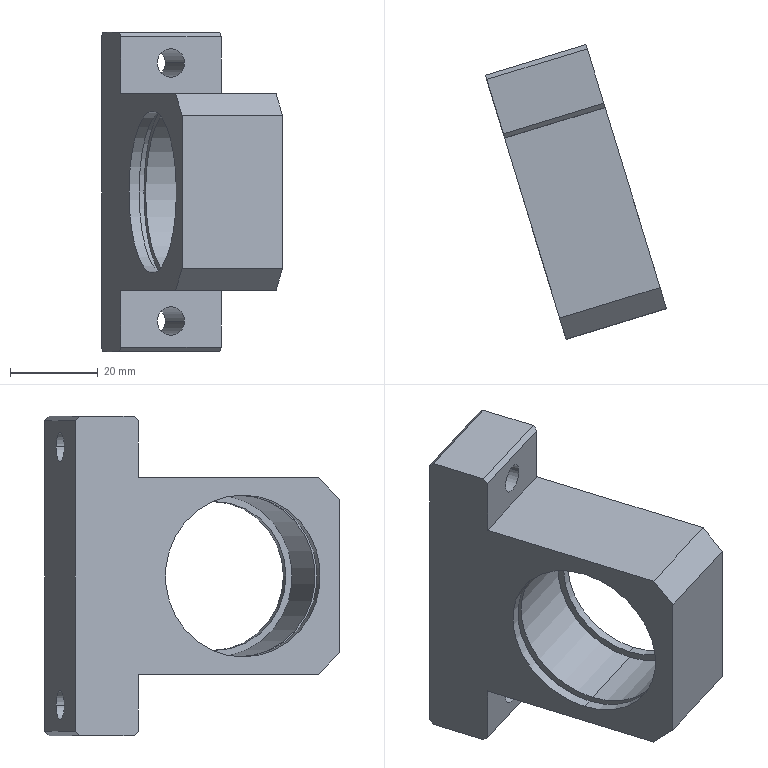Component | SolidWorks | v1ZHXTBGMWB6904ZZ_40SB1-1_V1ZHXTBearingMountingBaseSB1-1 | 1 solid | 31 faces | box 41.34 x 67.26 x 73 mm | volume 50736 mm3 | plane 19 | cylinder 12 | commonest cylinder face diameters 6.5 x4 37 x4 34 x2 39.8 x2
build123d program:
from build123d import *

# Parameters (mm, degrees)
BOSS_EXTRUDE1_DEPTH      = 12
BOSS_EXTRUDE1_DEPTH_BACK = 12
SKETCH3_R                = 3.25
CUT_EXTRUDE1_DEPTH       = 15
SKETCH4_R                = 3.25
CUT_EXTRUDE2_DEPTH       = 15
CHAMFER1_SIZE            = 5
CHAMFER2_SIZE            = 1


with BuildPart() as part:
    # Sketch1 → Boss-Extrude1 (new, two sides: drawn at the far end of the back side and taken through both)
    with BuildSketch(Plane.XY.offset(-BOSS_EXTRUDE1_DEPTH_BACK)):
        Polygon((-36.5, -40), (36.5, -40), (36.5, -25), (22.5, -25), (22.5, 23), (-22.5, 23), (-22.5, -25), (-36.5, -25), align=None)
    extrude(amount=BOSS_EXTRUDE1_DEPTH + BOSS_EXTRUDE1_DEPTH_BACK)

    # Sketch2 → Cut-Revolve1 (revolve, cut)
    with BuildSketch(Plane(origin=(0, 0, 0), x_dir=(0, 0, -1), z_dir=(1, 0, 0)), mode=Mode.PRIVATE) as cut_revolve1_sk:
        Polygon((-12, 0), (-12, 18.5), (-9.6, 18.5), (-9.6, 19.9), (-8, 19.9), (-8, 18.5), (10, 18.5), (10, 17), (12, 17), (12, 0), align=None)
    revolve(cut_revolve1_sk.sketch.rotate(Axis((0, 0, -12), (0, 0, 1)), 270), axis=Axis((0, 0, -12), (0, 0, 1)), mode=Mode.SUBTRACT)

    # Sketch3 → Cut-Extrude1 (cut)
    with BuildSketch(Plane(origin=(0, -40, 0), x_dir=(1, 0, 0), z_dir=(0, 1, 0))):
        with Locations(Location((-29.5, 0, 0), (0, 0, 270))):
            Circle(SKETCH3_R)
    extrude(amount=CUT_EXTRUDE1_DEPTH, mode=Mode.SUBTRACT)

    # Sketch4 → Cut-Extrude2 (cut)
    with BuildSketch(Plane(origin=(0, -40, 0), x_dir=(1, 0, 0), z_dir=(0, 1, 0))):
        with Locations(Location((29.5, 0, 0), (0, 0, 270))):
            Circle(SKETCH4_R)
    extrude(amount=CUT_EXTRUDE2_DEPTH, mode=Mode.SUBTRACT)

    # Chamfer1
    chamfer1_edges = [part.edges().sort_by_distance(p)[0] for p in [
        (-22.5, 23, 0),
        (22.5, 23, 0),
    ]]
    chamfer(chamfer1_edges, length=CHAMFER1_SIZE)

    # Chamfer2
    chamfer2_edges = [part.edges().sort_by_distance(p)[0] for p in [
        (-36.5, -25, 0),
        (36.5, -25, 0),
        (36.5, -40, 0),
        (-36.5, -40, 0),
    ]]
    chamfer(chamfer2_edges, length=CHAMFER2_SIZE)


solid = part.part

# Placed as in the assembly
solid = solid.moved(Location((165.24, -235.803, 375.239), (90, -73.032, -90)))
STEP:
#1=COLOUR_RGB('',0.7922,0.8196,0.9333);
#2=FILL_AREA_STYLE_COLOUR('',#1);
#3=FILL_AREA_STYLE('',(#2));
#4=SURFACE_STYLE_FILL_AREA(#3);
#5=SURFACE_SIDE_STYLE('',(#4));
#6=SURFACE_STYLE_USAGE(.BOTH.,#5);
#7=PRESENTATION_STYLE_ASSIGNMENT((#6));
#8=CARTESIAN_POINT('',(6.341,-8.305,13.612));
#9=VERTEX_POINT('',#8);
#10=CARTESIAN_POINT('',(6.096,-8.38,13.612));
#11=VERTEX_POINT('',#10);
#12=CARTESIAN_POINT('',(6.218,-8.342,13.612));
#13=DIRECTION('',(0.2918,-0.9565,-0.));
#14=DIRECTION('',(-0.9565,-0.2918,-0.));
#15=AXIS2_PLACEMENT_3D('',#12,#13,#14);
#16=CIRCLE('',#15,0.128);
#17=EDGE_CURVE('',#9,#11,#16,.T.);
#18=ORIENTED_EDGE('',*,*,#17,.T.);
#19=CARTESIAN_POINT('',(5.924,-7.815,13.612));
#20=VERTEX_POINT('',#19);
#21=CARTESIAN_POINT('',(6.096,-8.38,13.612));
#22=DIRECTION('',(-0.2918,0.9565,0.));
#23=VECTOR('',#22,39.37);
#24=LINE('',#21,#23);
#25=EDGE_CURVE('',#11,#20,#24,.T.);
#26=ORIENTED_EDGE('',*,*,#25,.T.);
#27=CARTESIAN_POINT('',(6.168,-7.74,13.612));
#28=VERTEX_POINT('',#27);
#29=CARTESIAN_POINT('',(6.046,-7.777,13.612));
#30=DIRECTION('',(0.2918,-0.9565,-0.));
#31=DIRECTION('',(-0.9565,-0.2918,-0.));
#32=AXIS2_PLACEMENT_3D('',#29,#30,#31);
#33=CIRCLE('',#32,0.128);
#34=EDGE_CURVE('',#28,#20,#33,.T.);
#35=ORIENTED_EDGE('',*,*,#34,.F.);
#36=CARTESIAN_POINT('',(6.341,-8.305,13.612));
#37=DIRECTION('',(-0.2918,0.9565,0.));
#38=VECTOR('',#37,39.37);
#39=LINE('',#36,#38);
#40=EDGE_CURVE('',#9,#28,#39,.T.);
#41=ORIENTED_EDGE('',*,*,#40,.F.);
#42=EDGE_LOOP('',(#18,#26,#35,#41));
#43=FACE_OUTER_BOUND('',#42,.T.);
#44=CARTESIAN_POINT('',(6.218,-8.342,13.612));
#45=DIRECTION('',(-0.2918,0.9565,0.));
#46=DIRECTION('',(0.9565,0.2918,0.));
#47=AXIS2_PLACEMENT_3D('',#44,#45,#46);
#48=CYLINDRICAL_SURFACE('',#47,0.128);
#49=ADVANCED_FACE('',(#43),#48,.F.);
#50=CARTESIAN_POINT('',(6.341,-8.305,15.935));
#51=VERTEX_POINT('',#50);
#52=CARTESIAN_POINT('',(6.096,-8.38,15.935));
#53=VERTEX_POINT('',#52);
#54=CARTESIAN_POINT('',(6.218,-8.342,15.935));
#55=DIRECTION('',(0.2918,-0.9565,-0.));
#56=DIRECTION('',(-0.9565,-0.2918,-0.));
#57=AXIS2_PLACEMENT_3D('',#54,#55,#56);
#58=CIRCLE('',#57,0.128);
#59=EDGE_CURVE('',#51,#53,#58,.T.);
#60=ORIENTED_EDGE('',*,*,#59,.T.);
#61=CARTESIAN_POINT('',(5.924,-7.815,15.935));
#62=VERTEX_POINT('',#61);
#63=CARTESIAN_POINT('',(6.096,-8.38,15.935));
#64=DIRECTION('',(-0.2918,0.9565,0.));
#65=VECTOR('',#64,39.37);
#66=LINE('',#63,#65);
#67=EDGE_CURVE('',#53,#62,#66,.T.);
#68=ORIENTED_EDGE('',*,*,#67,.T.);
#69=CARTESIAN_POINT('',(6.168,-7.74,15.935));
#70=VERTEX_POINT('',#69);
#71=CARTESIAN_POINT('',(6.046,-7.777,15.935));
#72=DIRECTION('',(0.2918,-0.9565,-0.));
#73=DIRECTION('',(-0.9565,-0.2918,-0.));
#74=AXIS2_PLACEMENT_3D('',#71,#72,#73);
#75=CIRCLE('',#74,0.128);
#76=EDGE_CURVE('',#70,#62,#75,.T.);
#77=ORIENTED_EDGE('',*,*,#76,.F.);
#78=CARTESIAN_POINT('',(6.341,-8.305,15.935));
#79=DIRECTION('',(-0.2918,0.9565,0.));
#80=VECTOR('',#79,39.37);
#81=LINE('',#78,#80);
#82=EDGE_CURVE('',#51,#70,#81,.T.);
#83=ORIENTED_EDGE('',*,*,#82,.F.);
#84=EDGE_LOOP('',(#60,#68,#77,#83));
#85=FACE_OUTER_BOUND('',#84,.T.);
#86=CARTESIAN_POINT('',(6.218,-8.342,15.935));
#87=DIRECTION('',(-0.2918,0.9565,0.));
#88=DIRECTION('',(0.9565,0.2918,0.));
#89=AXIS2_PLACEMENT_3D('',#86,#87,#88);
#90=CYLINDRICAL_SURFACE('',#89,0.128);
#91=ADVANCED_FACE('',(#85),#90,.F.);
#92=CARTESIAN_POINT('',(6.957,-9.146,15.442));
#93=VERTEX_POINT('',#92);
#94=CARTESIAN_POINT('',(6.957,-9.146,14.104));
#95=VERTEX_POINT('',#94);
#96=CARTESIAN_POINT('',(6.957,-9.146,14.773));
#97=DIRECTION('',(-0.9565,-0.2918,-0.));
#98=DIRECTION('',(0.,0.,-1.));
#99=AXIS2_PLACEMENT_3D('',#96,#97,#98);
#100=CIRCLE('',#99,0.6693);
#101=EDGE_CURVE('',#93,#95,#100,.T.);
#102=ORIENTED_EDGE('',*,*,#101,.F.);
#103=CARTESIAN_POINT('',(6.882,-9.169,15.442));
#104=VERTEX_POINT('',#103);
#105=CARTESIAN_POINT('',(6.957,-9.146,15.442));
#106=DIRECTION('',(-0.9565,-0.2918,-0.));
#107=VECTOR('',#106,39.37);
#108=LINE('',#105,#107);
#109=EDGE_CURVE('',#93,#104,#108,.T.);
#110=ORIENTED_EDGE('',*,*,#109,.T.);
#111=CARTESIAN_POINT('',(6.882,-9.169,14.104));
#112=VERTEX_POINT('',#111);
#113=CARTESIAN_POINT('',(6.882,-9.169,14.773));
#114=DIRECTION('',(-0.9565,-0.2918,-0.));
#115=DIRECTION('',(0.,0.,-1.));
#116=AXIS2_PLACEMENT_3D('',#113,#114,#115);
#117=CIRCLE('',#116,0.6693);
#118=EDGE_CURVE('',#104,#112,#117,.T.);
#119=ORIENTED_EDGE('',*,*,#118,.T.);
#120=CARTESIAN_POINT('',(6.957,-9.146,14.104));
#121=DIRECTION('',(-0.9565,-0.2918,-0.));
#122=VECTOR('',#121,39.37);
#123=LINE('',#120,#122);
#124=EDGE_CURVE('',#95,#112,#123,.T.);
#125=ORIENTED_EDGE('',*,*,#124,.F.);
#126=EDGE_LOOP('',(#102,#110,#119,#125));
#127=FACE_OUTER_BOUND('',#126,.T.);
#128=CARTESIAN_POINT('',(6.957,-9.146,14.773));
#129=DIRECTION('',(-0.9565,-0.2918,-0.));
#130=DIRECTION('',(0.,0.,-1.));
#131=AXIS2_PLACEMENT_3D('',#128,#129,#130);
#132=CYLINDRICAL_SURFACE('',#131,0.6693);
#133=ADVANCED_FACE('',(#127),#132,.F.);
#134=CARTESIAN_POINT('',(6.882,-9.169,15.502));
#135=VERTEX_POINT('',#134);
#136=CARTESIAN_POINT('',(6.882,-9.169,14.045));
#137=VERTEX_POINT('',#136);
#138=CARTESIAN_POINT('',(6.882,-9.169,14.773));
#139=DIRECTION('',(-0.9565,-0.2918,-0.));
#140=DIRECTION('',(0.,0.,-1.));
#141=AXIS2_PLACEMENT_3D('',#138,#139,#140);
#142=CIRCLE('',#141,0.7283);
#143=EDGE_CURVE('',#135,#137,#142,.T.);
#144=ORIENTED_EDGE('',*,*,#143,.F.);
#145=CARTESIAN_POINT('',(6.204,-9.375,15.502));
#146=VERTEX_POINT('',#145);
#147=CARTESIAN_POINT('',(6.957,-9.146,15.502));
#148=DIRECTION('',(-0.9565,-0.2918,-0.));
#149=VECTOR('',#148,39.37);
#150=LINE('',#147,#149);
#151=EDGE_CURVE('',#135,#146,#150,.T.);
#152=ORIENTED_EDGE('',*,*,#151,.T.);
#153=CARTESIAN_POINT('',(6.204,-9.375,14.045));
#154=VERTEX_POINT('',#153);
#155=CARTESIAN_POINT('',(6.204,-9.375,14.773));
#156=DIRECTION('',(-0.9565,-0.2918,-0.));
#157=DIRECTION('',(0.,0.,-1.));
#158=AXIS2_PLACEMENT_3D('',#155,#156,#157);
#159=CIRCLE('',#158,0.7283);
#160=EDGE_CURVE('',#146,#154,#159,.T.);
#161=ORIENTED_EDGE('',*,*,#160,.T.);
#162=CARTESIAN_POINT('',(6.957,-9.146,14.045));
#163=DIRECTION('',(-0.9565,-0.2918,-0.));
#164=VECTOR('',#163,39.37);
#165=LINE('',#162,#164);
#166=EDGE_CURVE('',#137,#154,#165,.T.);
#167=ORIENTED_EDGE('',*,*,#166,.F.);
#168=EDGE_LOOP('',(#144,#152,#161,#167));
#169=FACE_OUTER_BOUND('',#168,.T.);
#170=CARTESIAN_POINT('',(6.957,-9.146,14.773));
#171=DIRECTION('',(-0.9565,-0.2918,-0.));
#172=DIRECTION('',(0.,0.,-1.));
#173=AXIS2_PLACEMENT_3D('',#170,#171,#172);
#174=CYLINDRICAL_SURFACE('',#173,0.7283);
#175=ADVANCED_FACE('',(#169),#174,.F.);
#176=CARTESIAN_POINT('',(6.204,-9.375,15.557));
#177=VERTEX_POINT('',#176);
#178=CARTESIAN_POINT('',(6.204,-9.375,13.99));
#179=VERTEX_POINT('',#178);
#180=CARTESIAN_POINT('',(6.204,-9.375,14.773));
#181=DIRECTION('',(-0.9565,-0.2918,-0.));
#182=DIRECTION('',(0.,0.,-1.));
#183=AXIS2_PLACEMENT_3D('',#180,#181,#182);
#184=CIRCLE('',#183,0.7835);
#185=EDGE_CURVE('',#177,#179,#184,.T.);
#186=ORIENTED_EDGE('',*,*,#185,.F.);
#187=CARTESIAN_POINT('',(6.144,-9.394,15.557));
#188=VERTEX_POINT('',#187);
#189=CARTESIAN_POINT('',(6.957,-9.146,15.557));
#190=DIRECTION('',(-0.9565,-0.2918,-0.));
#191=VECTOR('',#190,39.37);
#192=LINE('',#189,#191);
#193=EDGE_CURVE('',#177,#188,#192,.T.);
#194=ORIENTED_EDGE('',*,*,#193,.T.);
#195=CARTESIAN_POINT('',(6.144,-9.394,13.99));
#196=VERTEX_POINT('',#195);
#197=CARTESIAN_POINT('',(6.144,-9.394,14.773));
#198=DIRECTION('',(-0.9565,-0.2918,-0.));
#199=DIRECTION('',(0.,0.,-1.));
#200=AXIS2_PLACEMENT_3D('',#197,#198,#199);
#201=CIRCLE('',#200,0.7835);
#202=EDGE_CURVE('',#188,#196,#201,.T.);
#203=ORIENTED_EDGE('',*,*,#202,.T.);
#204=CARTESIAN_POINT('',(6.957,-9.146,13.99));
#205=DIRECTION('',(-0.9565,-0.2918,-0.));
#206=VECTOR('',#205,39.37);
#207=LINE('',#204,#206);
#208=EDGE_CURVE('',#179,#196,#207,.T.);
#209=ORIENTED_EDGE('',*,*,#208,.F.);
#210=EDGE_LOOP('',(#186,#194,#203,#209));
#211=FACE_OUTER_BOUND('',#210,.T.);
#212=CARTESIAN_POINT('',(6.957,-9.146,14.773));
#213=DIRECTION('',(-0.9565,-0.2918,-0.));
#214=DIRECTION('',(0.,0.,-1.));
#215=AXIS2_PLACEMENT_3D('',#212,#213,#214);
#216=CYLINDRICAL_SURFACE('',#215,0.7835);
#217=ADVANCED_FACE('',(#211),#216,.F.);
#218=CARTESIAN_POINT('',(6.144,-9.394,15.502));
#219=VERTEX_POINT('',#218);
#220=CARTESIAN_POINT('',(6.144,-9.394,14.045));
#221=VERTEX_POINT('',#220);
#222=CARTESIAN_POINT('',(6.144,-9.394,14.773));
#223=DIRECTION('',(-0.9565,-0.2918,-0.));
#224=DIRECTION('',(0.,0.,-1.));
#225=AXIS2_PLACEMENT_3D('',#222,#223,#224);
#226=CIRCLE('',#225,0.7283);
#227=EDGE_CURVE('',#219,#221,#226,.T.);
#228=ORIENTED_EDGE('',*,*,#227,.F.);
#229=CARTESIAN_POINT('',(6.054,-9.421,15.502));
#230=VERTEX_POINT('',#229);
#231=CARTESIAN_POINT('',(6.957,-9.146,15.502));
#232=DIRECTION('',(-0.9565,-0.2918,-0.));
#233=VECTOR('',#232,39.37);
#234=LINE('',#231,#233);
#235=EDGE_CURVE('',#219,#230,#234,.T.);
#236=ORIENTED_EDGE('',*,*,#235,.T.);
#237=CARTESIAN_POINT('',(6.054,-9.421,14.045));
#238=VERTEX_POINT('',#237);
#239=CARTESIAN_POINT('',(6.054,-9.421,14.773));
#240=DIRECTION('',(-0.9565,-0.2918,-0.));
#241=DIRECTION('',(0.,0.,-1.));
#242=AXIS2_PLACEMENT_3D('',#239,#240,#241);
#243=CIRCLE('',#242,0.7283);
#244=EDGE_CURVE('',#230,#238,#243,.T.);
#245=ORIENTED_EDGE('',*,*,#244,.T.);
#246=CARTESIAN_POINT('',(6.957,-9.146,14.045));
#247=DIRECTION('',(-0.9565,-0.2918,-0.));
#248=VECTOR('',#247,39.37);
#249=LINE('',#246,#248);
#250=EDGE_CURVE('',#221,#238,#249,.T.);
#251=ORIENTED_EDGE('',*,*,#250,.F.);
#252=EDGE_LOOP('',(#228,#236,#245,#251));
#253=FACE_OUTER_BOUND('',#252,.T.);
#254=CARTESIAN_POINT('',(6.957,-9.146,14.773));
#255=DIRECTION('',(-0.9565,-0.2918,-0.));
#256=DIRECTION('',(0.,0.,-1.));
#257=AXIS2_PLACEMENT_3D('',#254,#255,#256);
#258=CYLINDRICAL_SURFACE('',#257,0.7283);
#259=ADVANCED_FACE('',(#253),#258,.F.);
#260=CARTESIAN_POINT('',(6.659,-8.167,16.21));
#261=VERTEX_POINT('',#260);
#262=CARTESIAN_POINT('',(6.509,-7.677,16.21));
#263=VERTEX_POINT('',#262);
#264=CARTESIAN_POINT('',(6.67,-8.204,16.21));
#265=DIRECTION('',(-0.2918,0.9565,0.));
#266=VECTOR('',#265,39.37);
#267=LINE('',#264,#266);
#268=EDGE_CURVE('',#261,#263,#267,.T.);
#269=ORIENTED_EDGE('',*,*,#268,.T.);
#270=CARTESIAN_POINT('',(5.606,-7.953,16.21));
#271=VERTEX_POINT('',#270);
#272=CARTESIAN_POINT('',(5.606,-7.953,16.21));
#273=DIRECTION('',(-0.9565,-0.2918,-0.));
#274=VECTOR('',#273,39.37);
#275=LINE('',#272,#274);
#276=EDGE_CURVE('',#263,#271,#275,.T.);
#277=ORIENTED_EDGE('',*,*,#276,.T.);
#278=CARTESIAN_POINT('',(5.755,-8.442,16.21));
#279=VERTEX_POINT('',#278);
#280=CARTESIAN_POINT('',(5.766,-8.48,16.21));
#281=DIRECTION('',(-0.2918,0.9565,0.));
#282=VECTOR('',#281,39.37);
#283=LINE('',#280,#282);
#284=EDGE_CURVE('',#279,#271,#283,.T.);
#285=ORIENTED_EDGE('',*,*,#284,.F.);
#286=CARTESIAN_POINT('',(5.755,-8.442,16.21));
#287=DIRECTION('',(0.9565,0.2918,0.));
#288=VECTOR('',#287,39.37);
#289=LINE('',#286,#288);
#290=EDGE_CURVE('',#279,#261,#289,.T.);
#291=ORIENTED_EDGE('',*,*,#290,.T.);
#292=EDGE_LOOP('',(#269,#277,#285,#291));
#293=FACE_OUTER_BOUND('',#292,.T.);
#294=CARTESIAN_POINT('',(5.766,-8.48,16.21));
#295=DIRECTION('',(0.,0.,-1.));
#296=DIRECTION('',(0.9565,0.2918,0.));
#297=AXIS2_PLACEMENT_3D('',#294,#295,#296);
#298=PLANE('',#297);
#299=ADVANCED_FACE('',(#293),#298,.F.);
#300=ORIENTED_EDGE('',*,*,#34,.T.);
#301=CARTESIAN_POINT('',(6.046,-7.777,13.612));
#302=DIRECTION('',(0.2918,-0.9565,-0.));
#303=DIRECTION('',(-0.9565,-0.2918,-0.));
#304=AXIS2_PLACEMENT_3D('',#301,#302,#303);
#305=CIRCLE('',#304,0.128);
#306=EDGE_CURVE('',#20,#28,#305,.T.);
#307=ORIENTED_EDGE('',*,*,#306,.T.);
#308=EDGE_LOOP('',(#300,#307));
#309=FACE_BOUND('',#308,.T.);
#310=ORIENTED_EDGE('',*,*,#76,.T.);
#311=CARTESIAN_POINT('',(6.046,-7.777,15.935));
#312=DIRECTION('',(0.2918,-0.9565,-0.));
#313=DIRECTION('',(-0.9565,-0.2918,-0.));
#314=AXIS2_PLACEMENT_3D('',#311,#312,#313);
#315=CIRCLE('',#314,0.128);
#316=EDGE_CURVE('',#62,#70,#315,.T.);
#317=ORIENTED_EDGE('',*,*,#316,.T.);
#318=EDGE_LOOP('',(#310,#317));
#319=FACE_BOUND('',#318,.T.);
#320=CARTESIAN_POINT('',(6.498,-7.639,16.171));
#321=VERTEX_POINT('',#320);
#322=CARTESIAN_POINT('',(6.498,-7.639,13.376));
#323=VERTEX_POINT('',#322);
#324=CARTESIAN_POINT('',(6.498,-7.639,16.21));
#325=DIRECTION('',(0.,0.,-1.));
#326=VECTOR('',#325,39.37);
#327=LINE('',#324,#326);
#328=EDGE_CURVE('',#321,#323,#327,.T.);
#329=ORIENTED_EDGE('',*,*,#328,.T.);
#330=CARTESIAN_POINT('',(5.594,-7.915,13.376));
#331=VERTEX_POINT('',#330);
#332=CARTESIAN_POINT('',(5.594,-7.915,13.376));
#333=DIRECTION('',(-0.9565,-0.2918,-0.));
#334=VECTOR('',#333,39.37);
#335=LINE('',#332,#334);
#336=EDGE_CURVE('',#323,#331,#335,.T.);
#337=ORIENTED_EDGE('',*,*,#336,.T.);
#338=CARTESIAN_POINT('',(5.594,-7.915,16.171));
#339=VERTEX_POINT('',#338);
#340=CARTESIAN_POINT('',(5.594,-7.915,16.21));
#341=DIRECTION('',(0.,0.,-1.));
#342=VECTOR('',#341,39.37);
#343=LINE('',#340,#342);
#344=EDGE_CURVE('',#339,#331,#343,.T.);
#345=ORIENTED_EDGE('',*,*,#344,.F.);
#346=CARTESIAN_POINT('',(5.594,-7.915,16.171));
#347=DIRECTION('',(0.9565,0.2918,0.));
#348=VECTOR('',#347,39.37);
#349=LINE('',#346,#348);
#350=EDGE_CURVE('',#339,#321,#349,.T.);
#351=ORIENTED_EDGE('',*,*,#350,.T.);
#352=EDGE_LOOP('',(#329,#337,#345,#351));
#353=FACE_OUTER_BOUND('',#352,.T.);
#354=CARTESIAN_POINT('',(5.594,-7.915,16.21));
#355=DIRECTION('',(0.2918,-0.9565,-0.));
#356=DIRECTION('',(-0.9565,-0.2918,-0.));
#357=AXIS2_PLACEMENT_3D('',#354,#355,#356);
#358=PLANE('',#357);
#359=ADVANCED_FACE('',(#309,#319,#353),#358,.F.);
#360=CARTESIAN_POINT('',(6.509,-7.677,13.336));
#361=VERTEX_POINT('',#360);
#362=CARTESIAN_POINT('',(6.659,-8.167,13.336));
#363=VERTEX_POINT('',#362);
#364=CARTESIAN_POINT('',(6.498,-7.639,13.336));
#365=DIRECTION('',(0.2918,-0.9565,-0.));
#366=VECTOR('',#365,39.37);
#367=LINE('',#364,#366);
#368=EDGE_CURVE('',#361,#363,#367,.T.);
#369=ORIENTED_EDGE('',*,*,#368,.T.);
#370=CARTESIAN_POINT('',(5.755,-8.442,13.336));
#371=VERTEX_POINT('',#370);
#372=CARTESIAN_POINT('',(5.755,-8.442,13.336));
#373=DIRECTION('',(-0.9565,-0.2918,-0.));
#374=VECTOR('',#373,39.37);
#375=LINE('',#372,#374);
#376=EDGE_CURVE('',#363,#371,#375,.T.);
#377=ORIENTED_EDGE('',*,*,#376,.T.);
#378=CARTESIAN_POINT('',(5.606,-7.953,13.336));
#379=VERTEX_POINT('',#378);
#380=CARTESIAN_POINT('',(5.594,-7.915,13.336));
#381=DIRECTION('',(0.2918,-0.9565,-0.));
#382=VECTOR('',#381,39.37);
#383=LINE('',#380,#382);
#384=EDGE_CURVE('',#379,#371,#383,.T.);
#385=ORIENTED_EDGE('',*,*,#384,.F.);
#386=CARTESIAN_POINT('',(5.606,-7.953,13.336));
#387=DIRECTION('',(0.9565,0.2918,0.));
#388=VECTOR('',#387,39.37);
#389=LINE('',#386,#388);
#390=EDGE_CURVE('',#379,#361,#389,.T.);
#391=ORIENTED_EDGE('',*,*,#390,.T.);
#392=EDGE_LOOP('',(#369,#377,#385,#391));
#393=FACE_OUTER_BOUND('',#392,.T.);
#394=CARTESIAN_POINT('',(5.594,-7.915,13.336));
#395=DIRECTION('',(-0.,-0.,1.));
#396=DIRECTION('',(-0.9565,-0.2918,-0.));
#397=AXIS2_PLACEMENT_3D('',#394,#395,#396);
#398=PLANE('',#397);
#399=ADVANCED_FACE('',(#393),#398,.F.);
#400=ORIENTED_EDGE('',*,*,#17,.F.);
#401=CARTESIAN_POINT('',(6.218,-8.342,13.612));
#402=DIRECTION('',(0.2918,-0.9565,-0.));
#403=DIRECTION('',(-0.9565,-0.2918,-0.));
#404=AXIS2_PLACEMENT_3D('',#401,#402,#403);
#405=CIRCLE('',#404,0.128);
#406=EDGE_CURVE('',#11,#9,#405,.T.);
#407=ORIENTED_EDGE('',*,*,#406,.F.);
#408=EDGE_LOOP('',(#400,#407));
#409=FACE_BOUND('',#408,.T.);
#410=CARTESIAN_POINT('',(5.766,-8.48,13.376));
#411=VERTEX_POINT('',#410);
#412=CARTESIAN_POINT('',(5.766,-8.48,13.887));
#413=VERTEX_POINT('',#412);
#414=CARTESIAN_POINT('',(5.766,-8.48,13.336));
#415=DIRECTION('',(-0.,-0.,1.));
#416=VECTOR('',#415,39.37);
#417=LINE('',#414,#416);
#418=EDGE_CURVE('',#411,#413,#417,.T.);
#419=ORIENTED_EDGE('',*,*,#418,.F.);
#420=CARTESIAN_POINT('',(6.67,-8.204,13.376));
#421=VERTEX_POINT('',#420);
#422=CARTESIAN_POINT('',(5.766,-8.48,13.376));
#423=DIRECTION('',(0.9565,0.2918,0.));
#424=VECTOR('',#423,39.37);
#425=LINE('',#422,#424);
#426=EDGE_CURVE('',#411,#421,#425,.T.);
#427=ORIENTED_EDGE('',*,*,#426,.T.);
#428=CARTESIAN_POINT('',(6.67,-8.204,13.887));
#429=VERTEX_POINT('',#428);
#430=CARTESIAN_POINT('',(6.67,-8.204,13.336));
#431=DIRECTION('',(-0.,-0.,1.));
#432=VECTOR('',#431,39.37);
#433=LINE('',#430,#432);
#434=EDGE_CURVE('',#421,#429,#433,.T.);
#435=ORIENTED_EDGE('',*,*,#434,.T.);
#436=CARTESIAN_POINT('',(5.766,-8.48,13.887));
#437=DIRECTION('',(0.9565,0.2918,0.));
#438=VECTOR('',#437,39.37);
#439=LINE('',#436,#438);
#440=EDGE_CURVE('',#413,#429,#439,.T.);
#441=ORIENTED_EDGE('',*,*,#440,.F.);
#442=EDGE_LOOP('',(#419,#427,#435,#441));
#443=FACE_OUTER_BOUND('',#442,.T.);
#444=CARTESIAN_POINT('',(5.766,-8.48,13.336));
#445=DIRECTION('',(-0.2918,0.9565,0.));
#446=DIRECTION('',(0.9565,0.2918,0.));
#447=AXIS2_PLACEMENT_3D('',#444,#445,#446);
#448=PLANE('',#447);
#449=ADVANCED_FACE('',(#409,#443),#448,.F.);
#450=CARTESIAN_POINT('',(7.164,-9.824,13.887));
#451=VERTEX_POINT('',#450);
#452=CARTESIAN_POINT('',(6.67,-8.204,13.887));
#453=DIRECTION('',(0.2918,-0.9565,-0.));
#454=VECTOR('',#453,39.37);
#455=LINE('',#452,#454);
#456=EDGE_CURVE('',#429,#451,#455,.T.);
#457=ORIENTED_EDGE('',*,*,#456,.T.);
#458=CARTESIAN_POINT('',(6.26,-10.099,13.887));
#459=VERTEX_POINT('',#458);
#460=CARTESIAN_POINT('',(6.26,-10.099,13.887));
#461=DIRECTION('',(-0.9565,-0.2918,-0.));
#462=VECTOR('',#461,39.37);
#463=LINE('',#460,#462);
#464=EDGE_CURVE('',#451,#459,#463,.T.);
#465=ORIENTED_EDGE('',*,*,#464,.T.);
#466=CARTESIAN_POINT('',(5.766,-8.48,13.887));
#467=DIRECTION('',(0.2918,-0.9565,-0.));
#468=VECTOR('',#467,39.37);
#469=LINE('',#466,#468);
#470=EDGE_CURVE('',#413,#459,#469,.T.);
#471=ORIENTED_EDGE('',*,*,#470,.F.);
#472=ORIENTED_EDGE('',*,*,#440,.T.);
#473=EDGE_LOOP('',(#457,#465,#471,#472));
#474=FACE_OUTER_BOUND('',#473,.T.);
#475=CARTESIAN_POINT('',(5.766,-8.48,13.887));
#476=DIRECTION('',(-0.,-0.,1.));
#477=DIRECTION('',(-0.9565,-0.2918,-0.));
#478=AXIS2_PLACEMENT_3D('',#475,#476,#477);
#479=PLANE('',#478);
#480=ADVANCED_FACE('',(#474),#479,.F.);
#481=CARTESIAN_POINT('',(7.222,-10.012,14.084));
#482=VERTEX_POINT('',#481);
#483=CARTESIAN_POINT('',(7.222,-10.012,15.462));
#484=VERTEX_POINT('',#483);
#485=CARTESIAN_POINT('',(7.222,-10.012,13.887));
#486=DIRECTION('',(-0.,-0.,1.));
#487=VECTOR('',#486,39.37);
#488=LINE('',#485,#487);
#489=EDGE_CURVE('',#482,#484,#488,.T.);
#490=ORIENTED_EDGE('',*,*,#489,.T.);
#491=CARTESIAN_POINT('',(6.318,-10.288,15.462));
#492=VERTEX_POINT('',#491);
#493=CARTESIAN_POINT('',(6.318,-10.288,15.462));
#494=DIRECTION('',(-0.9565,-0.2918,-0.));
#495=VECTOR('',#494,39.37);
#496=LINE('',#493,#495);
#497=EDGE_CURVE('',#484,#492,#496,.T.);
#498=ORIENTED_EDGE('',*,*,#497,.T.);
#499=CARTESIAN_POINT('',(6.318,-10.288,14.084));
#500=VERTEX_POINT('',#499);
#501=CARTESIAN_POINT('',(6.318,-10.288,13.887));
#502=DIRECTION('',(-0.,-0.,1.));
#503=VECTOR('',#502,39.37);
#504=LINE('',#501,#503);
#505=EDGE_CURVE('',#500,#492,#504,.T.);
#506=ORIENTED_EDGE('',*,*,#505,.F.);
#507=CARTESIAN_POINT('',(6.318,-10.288,14.084));
#508=DIRECTION('',(0.9565,0.2918,0.));
#509=VECTOR('',#508,39.37);
#510=LINE('',#507,#509);
#511=EDGE_CURVE('',#500,#482,#510,.T.);
#512=ORIENTED_EDGE('',*,*,#511,.T.);
#513=EDGE_LOOP('',(#490,#498,#506,#512));
#514=FACE_OUTER_BOUND('',#513,.T.);
#515=CARTESIAN_POINT('',(6.318,-10.288,13.887));
#516=DIRECTION('',(-0.2918,0.9565,0.));
#517=DIRECTION('',(0.9565,0.2918,0.));
#518=AXIS2_PLACEMENT_3D('',#515,#516,#517);
#519=PLANE('',#518);
#520=ADVANCED_FACE('',(#514),#519,.F.);
#521=CARTESIAN_POINT('',(6.26,-10.099,15.659));
#522=VERTEX_POINT('',#521);
#523=CARTESIAN_POINT('',(5.766,-8.48,15.659));
#524=VERTEX_POINT('',#523);
#525=CARTESIAN_POINT('',(6.318,-10.288,15.659));
#526=DIRECTION('',(-0.2918,0.9565,0.));
#527=VECTOR('',#526,39.37);
#528=LINE('',#525,#527);
#529=EDGE_CURVE('',#522,#524,#528,.T.);
#530=ORIENTED_EDGE('',*,*,#529,.F.);
#531=CARTESIAN_POINT('',(7.164,-9.824,15.659));
#532=VERTEX_POINT('',#531);
#533=CARTESIAN_POINT('',(6.26,-10.099,15.659));
#534=DIRECTION('',(0.9565,0.2918,0.));
#535=VECTOR('',#534,39.37);
#536=LINE('',#533,#535);
#537=EDGE_CURVE('',#522,#532,#536,.T.);
#538=ORIENTED_EDGE('',*,*,#537,.T.);
#539=CARTESIAN_POINT('',(6.67,-8.204,15.659));
#540=VERTEX_POINT('',#539);
#541=CARTESIAN_POINT('',(7.222,-10.012,15.659));
#542=DIRECTION('',(-0.2918,0.9565,0.));
#543=VECTOR('',#542,39.37);
#544=LINE('',#541,#543);
#545=EDGE_CURVE('',#532,#540,#544,.T.);
#546=ORIENTED_EDGE('',*,*,#545,.T.);
#547=CARTESIAN_POINT('',(5.766,-8.48,15.659));
#548=DIRECTION('',(0.9565,0.2918,0.));
#549=VECTOR('',#548,39.37);
#550=LINE('',#547,#549);
#551=EDGE_CURVE('',#524,#540,#550,.T.);
#552=ORIENTED_EDGE('',*,*,#551,.F.);
#553=EDGE_LOOP('',(#530,#538,#546,#552));
#554=FACE_OUTER_BOUND('',#553,.T.);
#555=CARTESIAN_POINT('',(6.318,-10.288,15.659));
#556=DIRECTION('',(0.,0.,-1.));
#557=DIRECTION('',(0.9565,0.2918,0.));
#558=AXIS2_PLACEMENT_3D('',#555,#556,#557);
#559=PLANE('',#558);
#560=ADVANCED_FACE('',(#554),#559,.F.);
#561=ORIENTED_EDGE('',*,*,#59,.F.);
#562=CARTESIAN_POINT('',(6.218,-8.342,15.935));
#563=DIRECTION('',(0.2918,-0.9565,-0.));
#564=DIRECTION('',(-0.9565,-0.2918,-0.));
#565=AXIS2_PLACEMENT_3D('',#562,#563,#564);
#566=CIRCLE('',#565,0.128);
#567=EDGE_CURVE('',#53,#51,#566,.T.);
#568=ORIENTED_EDGE('',*,*,#567,.F.);
#569=EDGE_LOOP('',(#561,#568));
#570=FACE_BOUND('',#569,.T.);
#571=CARTESIAN_POINT('',(6.67,-8.204,16.171));
#572=VERTEX_POINT('',#571);
#573=CARTESIAN_POINT('',(6.67,-8.204,15.659));
#574=DIRECTION('',(-0.,-0.,1.));
#575=VECTOR('',#574,39.37);
#576=LINE('',#573,#575);
#577=EDGE_CURVE('',#540,#572,#576,.T.);
#578=ORIENTED_EDGE('',*,*,#577,.T.);
#579=CARTESIAN_POINT('',(5.766,-8.48,16.171));
#580=VERTEX_POINT('',#579);
#581=CARTESIAN_POINT('',(5.766,-8.48,16.171));
#582=DIRECTION('',(-0.9565,-0.2918,-0.));
#583=VECTOR('',#582,39.37);
#584=LINE('',#581,#583);
#585=EDGE_CURVE('',#572,#580,#584,.T.);
#586=ORIENTED_EDGE('',*,*,#585,.T.);
#587=CARTESIAN_POINT('',(5.766,-8.48,15.659));
#588=DIRECTION('',(-0.,-0.,1.));
#589=VECTOR('',#588,39.37);
#590=LINE('',#587,#589);
#591=EDGE_CURVE('',#524,#580,#590,.T.);
#592=ORIENTED_EDGE('',*,*,#591,.F.);
#593=ORIENTED_EDGE('',*,*,#551,.T.);
#594=EDGE_LOOP('',(#578,#586,#592,#593));
#595=FACE_OUTER_BOUND('',#594,.T.);
#596=CARTESIAN_POINT('',(5.766,-8.48,15.659));
#597=DIRECTION('',(-0.2918,0.9565,0.));
#598=DIRECTION('',(0.9565,0.2918,0.));
#599=AXIS2_PLACEMENT_3D('',#596,#597,#598);
#600=PLANE('',#599);
#601=ADVANCED_FACE('',(#570,#595),#600,.F.);
#602=CARTESIAN_POINT('',(6.054,-9.421,14.773));
#603=DIRECTION('',(-0.9565,-0.2918,-0.));
#604=DIRECTION('',(0.,0.,-1.));
#605=AXIS2_PLACEMENT_3D('',#602,#603,#604);
#606=CIRCLE('',#605,0.7283);
#607=EDGE_CURVE('',#238,#230,#606,.T.);
#608=ORIENTED_EDGE('',*,*,#607,.F.);
#609=ORIENTED_EDGE('',*,*,#244,.F.);
#610=EDGE_LOOP('',(#608,#609));
#611=FACE_BOUND('',#610,.T.);
#612=ORIENTED_EDGE('',*,*,#384,.T.);
#613=CARTESIAN_POINT('',(6.114,-9.619,14.567));
#614=DIRECTION('',(0.2064,-0.6763,0.7071));
#615=VECTOR('',#614,39.37);
#616=LINE('',#613,#615);
#617=EDGE_CURVE('',#371,#411,#616,.T.);
#618=ORIENTED_EDGE('',*,*,#617,.T.);
#619=ORIENTED_EDGE('',*,*,#418,.T.);
#620=ORIENTED_EDGE('',*,*,#470,.T.);
#621=CARTESIAN_POINT('',(6.286,-10.184,13.976));
#622=DIRECTION('',(0.2064,-0.6763,0.7071));
#623=VECTOR('',#622,39.37);
#624=LINE('',#621,#623);
#625=EDGE_CURVE('',#459,#500,#624,.T.);
#626=ORIENTED_EDGE('',*,*,#625,.T.);
#627=ORIENTED_EDGE('',*,*,#505,.T.);
#628=CARTESIAN_POINT('',(6.286,-10.184,15.57));
#629=DIRECTION('',(-0.2064,0.6763,0.7071));
#630=VECTOR('',#629,39.37);
#631=LINE('',#628,#630);
#632=EDGE_CURVE('',#492,#522,#631,.T.);
#633=ORIENTED_EDGE('',*,*,#632,.T.);
#634=ORIENTED_EDGE('',*,*,#529,.T.);
#635=ORIENTED_EDGE('',*,*,#591,.T.);
#636=CARTESIAN_POINT('',(6.114,-9.619,14.98));
#637=DIRECTION('',(-0.2064,0.6763,0.7071));
#638=VECTOR('',#637,39.37);
#639=LINE('',#636,#638);
#640=EDGE_CURVE('',#580,#279,#639,.T.);
#641=ORIENTED_EDGE('',*,*,#640,.T.);
#642=ORIENTED_EDGE('',*,*,#284,.T.);
#643=CARTESIAN_POINT('',(5.62,-8.,16.259));
#644=DIRECTION('',(-0.2064,0.6763,-0.7071));
#645=VECTOR('',#644,39.37);
#646=LINE('',#643,#645);
#647=EDGE_CURVE('',#271,#339,#646,.T.);
#648=ORIENTED_EDGE('',*,*,#647,.T.);
#649=ORIENTED_EDGE('',*,*,#344,.T.);
#650=CARTESIAN_POINT('',(5.62,-8.,13.287));
#651=DIRECTION('',(0.2064,-0.6763,-0.7071));
#652=VECTOR('',#651,39.37);
#653=LINE('',#650,#652);
#654=EDGE_CURVE('',#331,#379,#653,.T.);
#655=ORIENTED_EDGE('',*,*,#654,.T.);
#656=EDGE_LOOP('',(#612,#618,#619,#620,#626,#627,#633,#634,#635,#641,#642,#648,#649,#655));
#657=FACE_OUTER_BOUND('',#656,.T.);
#658=CARTESIAN_POINT('',(6.054,-9.421,14.773));
#659=DIRECTION('',(-0.9565,-0.2918,-0.));
#660=DIRECTION('',(0.,0.,-1.));
#661=AXIS2_PLACEMENT_3D('',#658,#659,#660);
#662=PLANE('',#661);
#663=ADVANCED_FACE('',(#611,#657),#662,.T.);
#664=CARTESIAN_POINT('',(6.957,-9.146,14.773));
#665=DIRECTION('',(-0.9565,-0.2918,-0.));
#666=DIRECTION('',(0.,0.,-1.));
#667=AXIS2_PLACEMENT_3D('',#664,#665,#666);
#668=CIRCLE('',#667,0.6693);
#669=EDGE_CURVE('',#95,#93,#668,.T.);
#670=ORIENTED_EDGE('',*,*,#669,.T.);
#671=ORIENTED_EDGE('',*,*,#101,.T.);
#672=EDGE_LOOP('',(#670,#671));
#673=FACE_BOUND('',#672,.T.);
#674=ORIENTED_EDGE('',*,*,#434,.F.);
#675=CARTESIAN_POINT('',(6.67,-8.204,13.376));
#676=DIRECTION('',(-0.2064,0.6763,-0.7071));
#677=VECTOR('',#676,39.37);
#678=LINE('',#675,#677);
#679=EDGE_CURVE('',#421,#363,#678,.T.);
#680=ORIENTED_EDGE('',*,*,#679,.T.);
#681=ORIENTED_EDGE('',*,*,#368,.F.);
#682=CARTESIAN_POINT('',(6.509,-7.677,13.336));
#683=DIRECTION('',(-0.2064,0.6763,0.7071));
#684=VECTOR('',#683,39.37);
#685=LINE('',#682,#684);
#686=EDGE_CURVE('',#361,#323,#685,.T.);
#687=ORIENTED_EDGE('',*,*,#686,.T.);
#688=ORIENTED_EDGE('',*,*,#328,.F.);
#689=CARTESIAN_POINT('',(6.498,-7.639,16.171));
#690=DIRECTION('',(0.2064,-0.6763,0.7071));
#691=VECTOR('',#690,39.37);
#692=LINE('',#689,#691);
#693=EDGE_CURVE('',#321,#263,#692,.T.);
#694=ORIENTED_EDGE('',*,*,#693,.T.);
#695=ORIENTED_EDGE('',*,*,#268,.F.);
#696=CARTESIAN_POINT('',(6.659,-8.167,16.21));
#697=DIRECTION('',(0.2064,-0.6763,-0.7071));
#698=VECTOR('',#697,39.37);
#699=LINE('',#696,#698);
#700=EDGE_CURVE('',#261,#572,#699,.T.);
#701=ORIENTED_EDGE('',*,*,#700,.T.);
#702=ORIENTED_EDGE('',*,*,#577,.F.);
#703=ORIENTED_EDGE('',*,*,#545,.F.);
#704=CARTESIAN_POINT('',(7.164,-9.824,15.659));
#705=DIRECTION('',(0.2064,-0.6763,-0.7071));
#706=VECTOR('',#705,39.37);
#707=LINE('',#704,#706);
#708=EDGE_CURVE('',#532,#484,#707,.T.);
#709=ORIENTED_EDGE('',*,*,#708,.T.);
#710=ORIENTED_EDGE('',*,*,#489,.F.);
#711=CARTESIAN_POINT('',(7.222,-10.012,14.084));
#712=DIRECTION('',(-0.2064,0.6763,-0.7071));
#713=VECTOR('',#712,39.37);
#714=LINE('',#711,#713);
#715=EDGE_CURVE('',#482,#451,#714,.T.);
#716=ORIENTED_EDGE('',*,*,#715,.T.);
#717=ORIENTED_EDGE('',*,*,#456,.F.);
#718=EDGE_LOOP('',(#674,#680,#681,#687,#688,#694,#695,#701,#702,#703,#709,#710,#716,#717));
#719=FACE_OUTER_BOUND('',#718,.T.);
#720=CARTESIAN_POINT('',(6.957,-9.146,14.773));
#721=DIRECTION('',(-0.9565,-0.2918,-0.));
#722=DIRECTION('',(0.,0.,-1.));
#723=AXIS2_PLACEMENT_3D('',#720,#721,#722);
#724=PLANE('',#723);
#725=ADVANCED_FACE('',(#673,#719),#724,.F.);
#726=ORIENTED_EDGE('',*,*,#235,.F.);
#727=CARTESIAN_POINT('',(6.144,-9.394,14.773));
#728=DIRECTION('',(-0.9565,-0.2918,-0.));
#729=DIRECTION('',(0.,0.,-1.));
#730=AXIS2_PLACEMENT_3D('',#727,#728,#729);
#731=CIRCLE('',#730,0.7283);
#732=EDGE_CURVE('',#221,#219,#731,.T.);
#733=ORIENTED_EDGE('',*,*,#732,.F.);
#734=ORIENTED_EDGE('',*,*,#250,.T.);
#735=ORIENTED_EDGE('',*,*,#607,.T.);
#736=EDGE_LOOP('',(#726,#733,#734,#735));
#737=FACE_OUTER_BOUND('',#736,.T.);
#738=CARTESIAN_POINT('',(6.957,-9.146,14.773));
#739=DIRECTION('',(-0.9565,-0.2918,-0.));
#740=DIRECTION('',(0.,0.,-1.));
#741=AXIS2_PLACEMENT_3D('',#738,#739,#740);
#742=CYLINDRICAL_SURFACE('',#741,0.7283);
#743=ADVANCED_FACE('',(#737),#742,.F.);
#744=ORIENTED_EDGE('',*,*,#732,.T.);
#745=ORIENTED_EDGE('',*,*,#227,.T.);
#746=EDGE_LOOP('',(#744,#745));
#747=FACE_BOUND('',#746,.T.);
#748=CARTESIAN_POINT('',(6.144,-9.394,14.773));
#749=DIRECTION('',(-0.9565,-0.2918,-0.));
#750=DIRECTION('',(0.,0.,-1.));
#751=AXIS2_PLACEMENT_3D('',#748,#749,#750);
#752=CIRCLE('',#751,0.7835);
#753=EDGE_CURVE('',#196,#188,#752,.T.);
#754=ORIENTED_EDGE('',*,*,#753,.F.);
#755=ORIENTED_EDGE('',*,*,#202,.F.);
#756=EDGE_LOOP('',(#754,#755));
#757=FACE_OUTER_BOUND('',#756,.T.);
#758=CARTESIAN_POINT('',(6.357,-10.091,14.773));
#759=DIRECTION('',(0.9565,0.2918,0.));
#760=DIRECTION('',(-0.,-0.,1.));
#761=AXIS2_PLACEMENT_3D('',#758,#759,#760);
#762=PLANE('',#761);
#763=ADVANCED_FACE('',(#747,#757),#762,.T.);
#764=ORIENTED_EDGE('',*,*,#193,.F.);
#765=CARTESIAN_POINT('',(6.204,-9.375,14.773));
#766=DIRECTION('',(-0.9565,-0.2918,-0.));
#767=DIRECTION('',(0.,0.,-1.));
#768=AXIS2_PLACEMENT_3D('',#765,#766,#767);
#769=CIRCLE('',#768,0.7835);
#770=EDGE_CURVE('',#179,#177,#769,.T.);
#771=ORIENTED_EDGE('',*,*,#770,.F.);
#772=ORIENTED_EDGE('',*,*,#208,.T.);
#773=ORIENTED_EDGE('',*,*,#753,.T.);
#774=EDGE_LOOP('',(#764,#771,#772,#773));
#775=FACE_OUTER_BOUND('',#774,.T.);
#776=CARTESIAN_POINT('',(6.957,-9.146,14.773));
#777=DIRECTION('',(-0.9565,-0.2918,-0.));
#778=DIRECTION('',(0.,0.,-1.));
#779=AXIS2_PLACEMENT_3D('',#776,#777,#778);
#780=CYLINDRICAL_SURFACE('',#779,0.7835);
#781=ADVANCED_FACE('',(#775),#780,.F.);
#782=ORIENTED_EDGE('',*,*,#770,.T.);
#783=ORIENTED_EDGE('',*,*,#185,.T.);
#784=EDGE_LOOP('',(#782,#783));
#785=FACE_OUTER_BOUND('',#784,.T.);
#786=CARTESIAN_POINT('',(6.204,-9.375,14.773));
#787=DIRECTION('',(-0.9565,-0.2918,-0.));
#788=DIRECTION('',(0.,0.,-1.));
#789=AXIS2_PLACEMENT_3D('',#786,#787,#788);
#790=CIRCLE('',#789,0.7283);
#791=EDGE_CURVE('',#154,#146,#790,.T.);
#792=ORIENTED_EDGE('',*,*,#791,.F.);
#793=ORIENTED_EDGE('',*,*,#160,.F.);
#794=EDGE_LOOP('',(#792,#793));
#795=FACE_BOUND('',#794,.T.);
#796=CARTESIAN_POINT('',(6.433,-10.125,14.773));
#797=DIRECTION('',(-0.9565,-0.2918,-0.));
#798=DIRECTION('',(0.,0.,-1.));
#799=AXIS2_PLACEMENT_3D('',#796,#797,#798);
#800=PLANE('',#799);
#801=ADVANCED_FACE('',(#785,#795),#800,.T.);
#802=ORIENTED_EDGE('',*,*,#151,.F.);
#803=CARTESIAN_POINT('',(6.882,-9.169,14.773));
#804=DIRECTION('',(-0.9565,-0.2918,-0.));
#805=DIRECTION('',(0.,0.,-1.));
#806=AXIS2_PLACEMENT_3D('',#803,#804,#805);
#807=CIRCLE('',#806,0.7283);
#808=EDGE_CURVE('',#137,#135,#807,.T.);
#809=ORIENTED_EDGE('',*,*,#808,.F.);
#810=ORIENTED_EDGE('',*,*,#166,.T.);
#811=ORIENTED_EDGE('',*,*,#791,.T.);
#812=EDGE_LOOP('',(#802,#809,#810,#811));
#813=FACE_OUTER_BOUND('',#812,.T.);
#814=CARTESIAN_POINT('',(6.957,-9.146,14.773));
#815=DIRECTION('',(-0.9565,-0.2918,-0.));
#816=DIRECTION('',(0.,0.,-1.));
#817=AXIS2_PLACEMENT_3D('',#814,#815,#816);
#818=CYLINDRICAL_SURFACE('',#817,0.7283);
#819=ADVANCED_FACE('',(#813),#818,.F.);
#820=ORIENTED_EDGE('',*,*,#808,.T.);
#821=ORIENTED_EDGE('',*,*,#143,.T.);
#822=EDGE_LOOP('',(#820,#821));
#823=FACE_OUTER_BOUND('',#822,.T.);
#824=CARTESIAN_POINT('',(6.882,-9.169,14.773));
#825=DIRECTION('',(-0.9565,-0.2918,-0.));
#826=DIRECTION('',(0.,0.,-1.));
#827=AXIS2_PLACEMENT_3D('',#824,#825,#826);
#828=CIRCLE('',#827,0.6693);
#829=EDGE_CURVE('',#112,#104,#828,.T.);
#830=ORIENTED_EDGE('',*,*,#829,.F.);
#831=ORIENTED_EDGE('',*,*,#118,.F.);
#832=EDGE_LOOP('',(#830,#831));
#833=FACE_BOUND('',#832,.T.);
#834=CARTESIAN_POINT('',(7.095,-9.865,14.773));
#835=DIRECTION('',(-0.9565,-0.2918,-0.));
#836=DIRECTION('',(0.,0.,-1.));
#837=AXIS2_PLACEMENT_3D('',#834,#835,#836);
#838=PLANE('',#837);
#839=ADVANCED_FACE('',(#823,#833),#838,.T.);
#840=ORIENTED_EDGE('',*,*,#109,.F.);
#841=ORIENTED_EDGE('',*,*,#669,.F.);
#842=ORIENTED_EDGE('',*,*,#124,.T.);
#843=ORIENTED_EDGE('',*,*,#829,.T.);
#844=EDGE_LOOP('',(#840,#841,#842,#843));
#845=FACE_OUTER_BOUND('',#844,.T.);
#846=CARTESIAN_POINT('',(6.957,-9.146,14.773));
#847=DIRECTION('',(-0.9565,-0.2918,-0.));
#848=DIRECTION('',(0.,0.,-1.));
#849=AXIS2_PLACEMENT_3D('',#846,#847,#848);
#850=CYLINDRICAL_SURFACE('',#849,0.6693);
#851=ADVANCED_FACE('',(#845),#850,.F.);
#852=ORIENTED_EDGE('',*,*,#67,.F.);
#853=ORIENTED_EDGE('',*,*,#567,.T.);
#854=ORIENTED_EDGE('',*,*,#82,.T.);
#855=ORIENTED_EDGE('',*,*,#316,.F.);
#856=EDGE_LOOP('',(#852,#853,#854,#855));
#857=FACE_OUTER_BOUND('',#856,.T.);
#858=CARTESIAN_POINT('',(6.218,-8.342,15.935));
#859=DIRECTION('',(-0.2918,0.9565,0.));
#860=DIRECTION('',(0.9565,0.2918,0.));
#861=AXIS2_PLACEMENT_3D('',#858,#859,#860);
#862=CYLINDRICAL_SURFACE('',#861,0.128);
#863=ADVANCED_FACE('',(#857),#862,.F.);
#864=ORIENTED_EDGE('',*,*,#25,.F.);
#865=ORIENTED_EDGE('',*,*,#406,.T.);
#866=ORIENTED_EDGE('',*,*,#40,.T.);
#867=ORIENTED_EDGE('',*,*,#306,.F.);
#868=EDGE_LOOP('',(#864,#865,#866,#867));
#869=FACE_OUTER_BOUND('',#868,.T.);
#870=CARTESIAN_POINT('',(6.218,-8.342,13.612));
#871=DIRECTION('',(-0.2918,0.9565,0.));
#872=DIRECTION('',(0.9565,0.2918,0.));
#873=AXIS2_PLACEMENT_3D('',#870,#871,#872);
#874=CYLINDRICAL_SURFACE('',#873,0.128);
#875=ADVANCED_FACE('',(#869),#874,.F.);
#876=ORIENTED_EDGE('',*,*,#632,.F.);
#877=ORIENTED_EDGE('',*,*,#497,.F.);
#878=ORIENTED_EDGE('',*,*,#708,.F.);
#879=ORIENTED_EDGE('',*,*,#537,.F.);
#880=EDGE_LOOP('',(#876,#877,#878,#879));
#881=FACE_OUTER_BOUND('',#880,.T.);
#882=CARTESIAN_POINT('',(6.26,-10.099,15.659));
#883=DIRECTION('',(-0.2064,0.6763,-0.7071));
#884=DIRECTION('',(0.9565,0.2918,0.));
#885=AXIS2_PLACEMENT_3D('',#882,#883,#884);
#886=PLANE('',#885);
#887=ADVANCED_FACE('',(#881),#886,.F.);
#888=ORIENTED_EDGE('',*,*,#625,.F.);
#889=ORIENTED_EDGE('',*,*,#464,.F.);
#890=ORIENTED_EDGE('',*,*,#715,.F.);
#891=ORIENTED_EDGE('',*,*,#511,.F.);
#892=EDGE_LOOP('',(#888,#889,#890,#891));
#893=FACE_OUTER_BOUND('',#892,.T.);
#894=CARTESIAN_POINT('',(6.318,-10.288,14.084));
#895=DIRECTION('',(-0.2064,0.6763,0.7071));
#896=DIRECTION('',(0.9565,0.2918,0.));
#897=AXIS2_PLACEMENT_3D('',#894,#895,#896);
#898=PLANE('',#897);
#899=ADVANCED_FACE('',(#893),#898,.F.);
#900=ORIENTED_EDGE('',*,*,#617,.F.);
#901=ORIENTED_EDGE('',*,*,#376,.F.);
#902=ORIENTED_EDGE('',*,*,#679,.F.);
#903=ORIENTED_EDGE('',*,*,#426,.F.);
#904=EDGE_LOOP('',(#900,#901,#902,#903));
#905=FACE_OUTER_BOUND('',#904,.T.);
#906=CARTESIAN_POINT('',(5.766,-8.48,13.376));
#907=DIRECTION('',(-0.2064,0.6763,0.7071));
#908=DIRECTION('',(0.9565,0.2918,0.));
#909=AXIS2_PLACEMENT_3D('',#906,#907,#908);
#910=PLANE('',#909);
#911=ADVANCED_FACE('',(#905),#910,.F.);
#912=ORIENTED_EDGE('',*,*,#654,.F.);
#913=ORIENTED_EDGE('',*,*,#336,.F.);
#914=ORIENTED_EDGE('',*,*,#686,.F.);
#915=ORIENTED_EDGE('',*,*,#390,.F.);
#916=EDGE_LOOP('',(#912,#913,#914,#915));
#917=FACE_OUTER_BOUND('',#916,.T.);
#918=CARTESIAN_POINT('',(5.606,-7.953,13.336));
#919=DIRECTION('',(0.2064,-0.6763,0.7071));
#920=DIRECTION('',(0.9565,0.2918,0.));
#921=AXIS2_PLACEMENT_3D('',#918,#919,#920);
#922=PLANE('',#921);
#923=ADVANCED_FACE('',(#917),#922,.F.);
#924=ORIENTED_EDGE('',*,*,#647,.F.);
#925=ORIENTED_EDGE('',*,*,#276,.F.);
#926=ORIENTED_EDGE('',*,*,#693,.F.);
#927=ORIENTED_EDGE('',*,*,#350,.F.);
#928=EDGE_LOOP('',(#924,#925,#926,#927));
#929=FACE_OUTER_BOUND('',#928,.T.);
#930=CARTESIAN_POINT('',(5.594,-7.915,16.171));
#931=DIRECTION('',(0.2064,-0.6763,-0.7071));
#932=DIRECTION('',(0.9565,0.2918,0.));
#933=AXIS2_PLACEMENT_3D('',#930,#931,#932);
#934=PLANE('',#933);
#935=ADVANCED_FACE('',(#929),#934,.F.);
#936=ORIENTED_EDGE('',*,*,#640,.F.);
#937=ORIENTED_EDGE('',*,*,#585,.F.);
#938=ORIENTED_EDGE('',*,*,#700,.F.);
#939=ORIENTED_EDGE('',*,*,#290,.F.);
#940=EDGE_LOOP('',(#936,#937,#938,#939));
#941=FACE_OUTER_BOUND('',#940,.T.);
#942=CARTESIAN_POINT('',(5.755,-8.442,16.21));
#943=DIRECTION('',(-0.2064,0.6763,-0.7071));
#944=DIRECTION('',(0.9565,0.2918,0.));
#945=AXIS2_PLACEMENT_3D('',#942,#943,#944);
#946=PLANE('',#945);
#947=ADVANCED_FACE('',(#941),#946,.F.);
#948=CLOSED_SHELL('',(#49,#91,#133,#175,#217,#259,#299,#359,#399,#449,#480,#520,#560,#601,#663,#725,#743,#763,#781,#801,#819,#839,#851,#863,#875,#887,#899,#911,#923,#935,#947));
#949=MANIFOLD_SOLID_BREP('',#948);
#950=STYLED_ITEM('',(#7),#949);
#951=(LENGTH_UNIT()NAMED_UNIT(*)SI_UNIT($,.METRE.));
#952=LENGTH_MEASURE_WITH_UNIT(LENGTH_MEASURE(0.0254),#951);
#953=DIMENSIONAL_EXPONENTS(1.,0.,0.,0.,0.,0.,0.);
#954=(CONVERSION_BASED_UNIT('',#952)LENGTH_UNIT()NAMED_UNIT(#953));
#955=UNCERTAINTY_MEASURE_WITH_UNIT(LENGTH_MEASURE(0.00001),#954,'','');
#956=(NAMED_UNIT(*)PLANE_ANGLE_UNIT()SI_UNIT($,.RADIAN.));
#957=(NAMED_UNIT(*)SI_UNIT($,.STERADIAN.)SOLID_ANGLE_UNIT());
#958=(GEOMETRIC_REPRESENTATION_CONTEXT(3)GLOBAL_UNCERTAINTY_ASSIGNED_CONTEXT((#955))GLOBAL_UNIT_ASSIGNED_CONTEXT((#954,#956,#957))REPRESENTATION_CONTEXT('',''));
#959=MECHANICAL_DESIGN_GEOMETRIC_PRESENTATION_REPRESENTATION('',(#950),#958);
#960=PRESENTATION_LAYER_ASSIGNMENT('','',(#950));
#961=CARTESIAN_POINT('',(0.,0.,0.));
#962=DIRECTION('',(0.,0.,1.));
#963=DIRECTION('',(1.,0.,0.));
#964=AXIS2_PLACEMENT_3D('',#961,#962,#963);
#965=(LENGTH_UNIT()NAMED_UNIT(*)SI_UNIT($,.METRE.));
#966=LENGTH_MEASURE_WITH_UNIT(LENGTH_MEASURE(0.0254),#965);
#967=DIMENSIONAL_EXPONENTS(1.,0.,0.,0.,0.,0.,0.);
#968=(CONVERSION_BASED_UNIT('',#966)LENGTH_UNIT()NAMED_UNIT(#967));
#969=UNCERTAINTY_MEASURE_WITH_UNIT(LENGTH_MEASURE(0.00001),#968,'','');
#970=(NAMED_UNIT(*)PLANE_ANGLE_UNIT()SI_UNIT($,.RADIAN.));
#971=(NAMED_UNIT(*)SI_UNIT($,.STERADIAN.)SOLID_ANGLE_UNIT());
#972=(GEOMETRIC_REPRESENTATION_CONTEXT(3)GLOBAL_UNCERTAINTY_ASSIGNED_CONTEXT((#969))GLOBAL_UNIT_ASSIGNED_CONTEXT((#968,#970,#971))REPRESENTATION_CONTEXT('',''));
#973=ADVANCED_BREP_SHAPE_REPRESENTATION('',(#949,#964),#972);